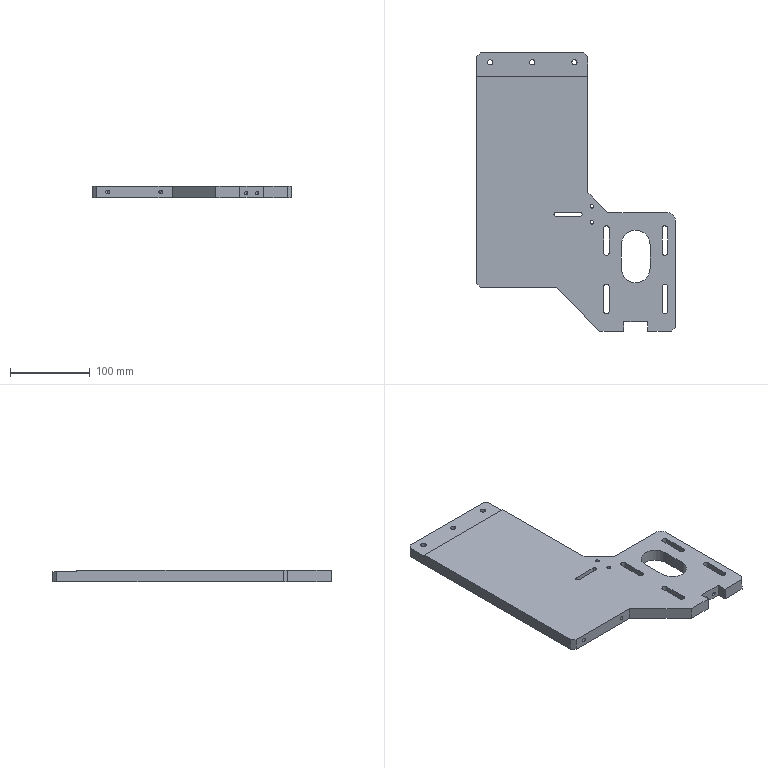Component | SolidWorks | XT-1-12-2-1 | 1 solid | 88 faces | volume 811672 mm3 | cylinder 42 | plane 38 | cone 8 | commonest cylinder face diameters 7 x8 11 x6 6.6 x6 8 x4 4.5 x4 5 x4 4.2 x4 5.3 x3